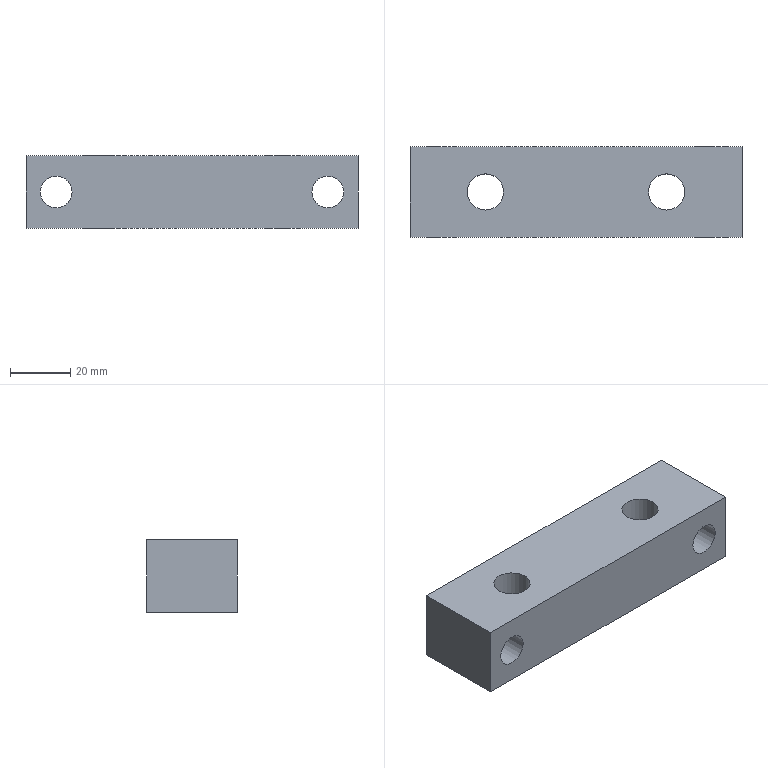Component | NX | SUPPORT_BLOCK | 1 solid | 10 faces | box 110 x 30 x 24 mm | volume 68576 mm3 | plane 6 | cylinder 4 | commonest cylinder face diameters 12 x2 10.5 x2
STEP:
#1=CARTESIAN_POINT('',(0.,0.,0.));
#2=DIRECTION('',(0.,0.,1.));
#3=DIRECTION('',(1.,0.,0.));
#4=AXIS2_PLACEMENT_3D('',#1,#2,#3);
#5=CARTESIAN_POINT('',(-25.,-15.,225.));
#6=VERTEX_POINT('',#5);
#7=CARTESIAN_POINT('',(-25.,15.,225.));
#8=VERTEX_POINT('',#7);
#9=CARTESIAN_POINT('',(-25.,-15.,225.));
#10=DIRECTION('',(0.,1.,0.));
#11=VECTOR('',#10,1.);
#12=LINE('',#9,#11);
#13=CARTESIAN_POINT('',(-25.,-15.,201.));
#14=DIRECTION('',(1.,0.,0.));
#15=DIRECTION('',(0.,1.,0.));
#16=AXIS2_PLACEMENT_3D('',#13,#14,#15);
#17=PLANE('',#16);
#18=CARTESIAN_POINT('',(0.,24.));
#19=DIRECTION('',(1.,0.));
#20=VECTOR('',#19,1.);
#21=LINE('',#18,#20);
#22=(GEOMETRIC_REPRESENTATION_CONTEXT(2)PARAMETRIC_REPRESENTATION_CONTEXT()REPRESENTATION_CONTEXT('',''));
#23=DEFINITIONAL_REPRESENTATION('',(#21),#22);
#24=PCURVE('',#17,#23);
#25=CARTESIAN_POINT('',(0.,0.,225.));
#26=DIRECTION('',(0.,0.,1.));
#27=DIRECTION('',(0.,-1.,0.));
#28=AXIS2_PLACEMENT_3D('',#25,#26,#27);
#29=PLANE('',#28);
#30=CARTESIAN_POINT('',(15.,-25.));
#31=DIRECTION('',(-1.,0.));
#32=VECTOR('',#31,1.);
#33=LINE('',#30,#32);
#34=(GEOMETRIC_REPRESENTATION_CONTEXT(2)PARAMETRIC_REPRESENTATION_CONTEXT()REPRESENTATION_CONTEXT('',''));
#35=DEFINITIONAL_REPRESENTATION('',(#33),#34);
#36=PCURVE('',#29,#35);
#37=SURFACE_CURVE('',#12,(#24,#36),.PCURVE_S1.);
#38=EDGE_CURVE('',#6,#8,#37,.T.);
#39=ORIENTED_EDGE('',*,*,#38,.T.);
#40=CARTESIAN_POINT('',(-25.,15.,201.));
#41=VERTEX_POINT('',#40);
#42=CARTESIAN_POINT('',(-25.,15.,201.));
#43=DIRECTION('',(0.,0.,1.));
#44=VECTOR('',#43,1.);
#45=LINE('',#42,#44);
#46=CARTESIAN_POINT('',(30.,0.));
#47=DIRECTION('',(0.,1.));
#48=VECTOR('',#47,1.);
#49=LINE('',#46,#48);
#50=(GEOMETRIC_REPRESENTATION_CONTEXT(2)PARAMETRIC_REPRESENTATION_CONTEXT()REPRESENTATION_CONTEXT('',''));
#51=DEFINITIONAL_REPRESENTATION('',(#49),#50);
#52=PCURVE('',#17,#51);
#53=CARTESIAN_POINT('',(-25.,15.,201.));
#54=DIRECTION('',(0.,-1.,0.));
#55=DIRECTION('',(1.,0.,0.));
#56=AXIS2_PLACEMENT_3D('',#53,#54,#55);
#57=PLANE('',#56);
#58=CARTESIAN_POINT('',(0.,0.));
#59=DIRECTION('',(0.,1.));
#60=VECTOR('',#59,1.);
#61=LINE('',#58,#60);
#62=(GEOMETRIC_REPRESENTATION_CONTEXT(2)PARAMETRIC_REPRESENTATION_CONTEXT()REPRESENTATION_CONTEXT('',''));
#63=DEFINITIONAL_REPRESENTATION('',(#61),#62);
#64=PCURVE('',#57,#63);
#65=SURFACE_CURVE('',#45,(#52,#64),.PCURVE_S1.);
#66=EDGE_CURVE('',#41,#8,#65,.T.);
#67=ORIENTED_EDGE('',*,*,#66,.F.);
#68=CARTESIAN_POINT('',(-25.,-15.,201.));
#69=VERTEX_POINT('',#68);
#70=CARTESIAN_POINT('',(-25.,-15.,201.));
#71=DIRECTION('',(0.,1.,0.));
#72=VECTOR('',#71,1.);
#73=LINE('',#70,#72);
#74=CARTESIAN_POINT('',(0.,0.));
#75=DIRECTION('',(1.,0.));
#76=VECTOR('',#75,1.);
#77=LINE('',#74,#76);
#78=(GEOMETRIC_REPRESENTATION_CONTEXT(2)PARAMETRIC_REPRESENTATION_CONTEXT()REPRESENTATION_CONTEXT('',''));
#79=DEFINITIONAL_REPRESENTATION('',(#77),#78);
#80=PCURVE('',#17,#79);
#81=CARTESIAN_POINT('',(0.,0.,201.));
#82=DIRECTION('',(0.,0.,1.));
#83=DIRECTION('',(0.,-1.,0.));
#84=AXIS2_PLACEMENT_3D('',#81,#82,#83);
#85=PLANE('',#84);
#86=CARTESIAN_POINT('',(15.,-25.));
#87=DIRECTION('',(-1.,0.));
#88=VECTOR('',#87,1.);
#89=LINE('',#86,#88);
#90=(GEOMETRIC_REPRESENTATION_CONTEXT(2)PARAMETRIC_REPRESENTATION_CONTEXT()REPRESENTATION_CONTEXT('',''));
#91=DEFINITIONAL_REPRESENTATION('',(#89),#90);
#92=PCURVE('',#85,#91);
#93=SURFACE_CURVE('',#73,(#80,#92),.PCURVE_S1.);
#94=EDGE_CURVE('',#69,#41,#93,.T.);
#95=ORIENTED_EDGE('',*,*,#94,.F.);
#96=CARTESIAN_POINT('',(-25.,-15.,201.));
#97=DIRECTION('',(0.,0.,1.));
#98=VECTOR('',#97,1.);
#99=LINE('',#96,#98);
#100=CARTESIAN_POINT('',(0.,0.));
#101=DIRECTION('',(0.,1.));
#102=VECTOR('',#101,1.);
#103=LINE('',#100,#102);
#104=(GEOMETRIC_REPRESENTATION_CONTEXT(2)PARAMETRIC_REPRESENTATION_CONTEXT()REPRESENTATION_CONTEXT('',''));
#105=DEFINITIONAL_REPRESENTATION('',(#103),#104);
#106=PCURVE('',#17,#105);
#107=CARTESIAN_POINT('',(85.,-15.,201.));
#108=DIRECTION('',(-0.,1.,0.));
#109=DIRECTION('',(-1.,-0.,0.));
#110=AXIS2_PLACEMENT_3D('',#107,#108,#109);
#111=PLANE('',#110);
#112=CARTESIAN_POINT('',(110.,0.));
#113=DIRECTION('',(0.,1.));
#114=VECTOR('',#113,1.);
#115=LINE('',#112,#114);
#116=(GEOMETRIC_REPRESENTATION_CONTEXT(2)PARAMETRIC_REPRESENTATION_CONTEXT()REPRESENTATION_CONTEXT('',''));
#117=DEFINITIONAL_REPRESENTATION('',(#115),#116);
#118=PCURVE('',#111,#117);
#119=SURFACE_CURVE('',#99,(#106,#118),.PCURVE_S1.);
#120=EDGE_CURVE('',#69,#6,#119,.T.);
#121=ORIENTED_EDGE('',*,*,#120,.T.);
#122=EDGE_LOOP('',(#39,#67,#95,#121));
#123=FACE_BOUND('',#122,.T.);
#124=ADVANCED_FACE('',(#123),#17,.F.);
#125=CARTESIAN_POINT('',(-9.75,15.,213.));
#126=VERTEX_POINT('',#125);
#127=CARTESIAN_POINT('',(-15.,15.,213.));
#128=DIRECTION('',(-0.,1.,0.));
#129=DIRECTION('',(1.,0.,0.));
#130=AXIS2_PLACEMENT_3D('',#127,#128,#129);
#131=CIRCLE('',#130,5.25);
#132=CARTESIAN_POINT('',(15.25,12.));
#133=CARTESIAN_POINT('',(15.25,2.907));
#134=CARTESIAN_POINT('',(7.375,7.453));
#135=CARTESIAN_POINT('',(-0.5,12.));
#136=CARTESIAN_POINT('',(7.375,16.547));
#137=CARTESIAN_POINT('',(15.25,21.093));
#138=CARTESIAN_POINT('',(15.25,12.));
#139=(BOUNDED_CURVE()B_SPLINE_CURVE(2,(#132,#133,#134,#135,#136,#137,#138),.UNSPECIFIED.,.T.,.F.)B_SPLINE_CURVE_WITH_KNOTS((1,2,2,2,2,1),(-2.094,0.,2.094,4.189,6.283,8.378),.UNSPECIFIED.)CURVE()GEOMETRIC_REPRESENTATION_ITEM()RATIONAL_B_SPLINE_CURVE((1.,0.5,1.,0.5,1.,0.5,1.))REPRESENTATION_ITEM(''));
#140=(GEOMETRIC_REPRESENTATION_CONTEXT(2)PARAMETRIC_REPRESENTATION_CONTEXT()REPRESENTATION_CONTEXT('',''));
#141=DEFINITIONAL_REPRESENTATION('',(#139),#140);
#142=PCURVE('',#57,#141);
#143=CARTESIAN_POINT('',(-15.,22.,213.));
#144=DIRECTION('',(0.,-1.,0.));
#145=DIRECTION('',(1.,0.,0.));
#146=AXIS2_PLACEMENT_3D('',#143,#144,#145);
#147=CYLINDRICAL_SURFACE('',#146,5.25);
#148=CARTESIAN_POINT('',(6.283,7.));
#149=DIRECTION('',(-1.,0.));
#150=VECTOR('',#149,1.);
#151=LINE('',#148,#150);
#152=(GEOMETRIC_REPRESENTATION_CONTEXT(2)PARAMETRIC_REPRESENTATION_CONTEXT()REPRESENTATION_CONTEXT('',''));
#153=DEFINITIONAL_REPRESENTATION('',(#151),#152);
#154=PCURVE('',#147,#153);
#155=SURFACE_CURVE('',#131,(#142,#154),.PCURVE_S1.);
#156=EDGE_CURVE('',#126,#126,#155,.T.);
#157=ORIENTED_EDGE('',*,*,#156,.F.);
#158=EDGE_LOOP('',(#157));
#159=FACE_BOUND('',#158,.T.);
#160=CARTESIAN_POINT('',(80.25,15.,213.));
#161=VERTEX_POINT('',#160);
#162=CARTESIAN_POINT('',(75.,15.,213.));
#163=DIRECTION('',(0.,-1.,0.));
#164=DIRECTION('',(1.,0.,0.));
#165=AXIS2_PLACEMENT_3D('',#162,#163,#164);
#166=CIRCLE('',#165,5.25);
#167=CARTESIAN_POINT('',(100.,12.));
#168=DIRECTION('',(1.,0.));
#169=AXIS2_PLACEMENT_2D('',#167,#168);
#170=CIRCLE('',#169,5.25);
#171=(GEOMETRIC_REPRESENTATION_CONTEXT(2)PARAMETRIC_REPRESENTATION_CONTEXT()REPRESENTATION_CONTEXT('',''));
#172=DEFINITIONAL_REPRESENTATION('',(#170),#171);
#173=PCURVE('',#57,#172);
#174=CARTESIAN_POINT('',(75.,22.,213.));
#175=DIRECTION('',(0.,-1.,0.));
#176=DIRECTION('',(1.,0.,0.));
#177=AXIS2_PLACEMENT_3D('',#174,#175,#176);
#178=CYLINDRICAL_SURFACE('',#177,5.25);
#179=CARTESIAN_POINT('',(0.,7.));
#180=DIRECTION('',(1.,0.));
#181=VECTOR('',#180,1.);
#182=LINE('',#179,#181);
#183=(GEOMETRIC_REPRESENTATION_CONTEXT(2)PARAMETRIC_REPRESENTATION_CONTEXT()REPRESENTATION_CONTEXT('',''));
#184=DEFINITIONAL_REPRESENTATION('',(#182),#183);
#185=PCURVE('',#178,#184);
#186=SURFACE_CURVE('',#166,(#173,#185),.PCURVE_S1.);
#187=EDGE_CURVE('',#161,#161,#186,.T.);
#188=ORIENTED_EDGE('',*,*,#187,.T.);
#189=EDGE_LOOP('',(#188));
#190=FACE_BOUND('',#189,.T.);
#191=CARTESIAN_POINT('',(85.,15.,225.));
#192=VERTEX_POINT('',#191);
#193=CARTESIAN_POINT('',(-25.,15.,225.));
#194=DIRECTION('',(1.,0.,0.));
#195=VECTOR('',#194,1.);
#196=LINE('',#193,#195);
#197=CARTESIAN_POINT('',(0.,24.));
#198=DIRECTION('',(1.,0.));
#199=VECTOR('',#198,1.);
#200=LINE('',#197,#199);
#201=(GEOMETRIC_REPRESENTATION_CONTEXT(2)PARAMETRIC_REPRESENTATION_CONTEXT()REPRESENTATION_CONTEXT('',''));
#202=DEFINITIONAL_REPRESENTATION('',(#200),#201);
#203=PCURVE('',#57,#202);
#204=CARTESIAN_POINT('',(-15.,-25.));
#205=DIRECTION('',(-0.,1.));
#206=VECTOR('',#205,1.);
#207=LINE('',#204,#206);
#208=(GEOMETRIC_REPRESENTATION_CONTEXT(2)PARAMETRIC_REPRESENTATION_CONTEXT()REPRESENTATION_CONTEXT('',''));
#209=DEFINITIONAL_REPRESENTATION('',(#207),#208);
#210=PCURVE('',#29,#209);
#211=SURFACE_CURVE('',#196,(#203,#210),.PCURVE_S1.);
#212=EDGE_CURVE('',#8,#192,#211,.T.);
#213=ORIENTED_EDGE('',*,*,#212,.T.);
#214=CARTESIAN_POINT('',(85.,15.,201.));
#215=VERTEX_POINT('',#214);
#216=CARTESIAN_POINT('',(85.,15.,201.));
#217=DIRECTION('',(0.,0.,1.));
#218=VECTOR('',#217,1.);
#219=LINE('',#216,#218);
#220=CARTESIAN_POINT('',(110.,0.));
#221=DIRECTION('',(0.,1.));
#222=VECTOR('',#221,1.);
#223=LINE('',#220,#222);
#224=(GEOMETRIC_REPRESENTATION_CONTEXT(2)PARAMETRIC_REPRESENTATION_CONTEXT()REPRESENTATION_CONTEXT('',''));
#225=DEFINITIONAL_REPRESENTATION('',(#223),#224);
#226=PCURVE('',#57,#225);
#227=CARTESIAN_POINT('',(85.,15.,201.));
#228=DIRECTION('',(-1.,-0.,0.));
#229=DIRECTION('',(0.,-1.,0.));
#230=AXIS2_PLACEMENT_3D('',#227,#228,#229);
#231=PLANE('',#230);
#232=CARTESIAN_POINT('',(0.,0.));
#233=DIRECTION('',(0.,1.));
#234=VECTOR('',#233,1.);
#235=LINE('',#232,#234);
#236=(GEOMETRIC_REPRESENTATION_CONTEXT(2)PARAMETRIC_REPRESENTATION_CONTEXT()REPRESENTATION_CONTEXT('',''));
#237=DEFINITIONAL_REPRESENTATION('',(#235),#236);
#238=PCURVE('',#231,#237);
#239=SURFACE_CURVE('',#219,(#226,#238),.PCURVE_S1.);
#240=EDGE_CURVE('',#215,#192,#239,.T.);
#241=ORIENTED_EDGE('',*,*,#240,.F.);
#242=CARTESIAN_POINT('',(-25.,15.,201.));
#243=DIRECTION('',(1.,0.,0.));
#244=VECTOR('',#243,1.);
#245=LINE('',#242,#244);
#246=CARTESIAN_POINT('',(0.,0.));
#247=DIRECTION('',(1.,0.));
#248=VECTOR('',#247,1.);
#249=LINE('',#246,#248);
#250=(GEOMETRIC_REPRESENTATION_CONTEXT(2)PARAMETRIC_REPRESENTATION_CONTEXT()REPRESENTATION_CONTEXT('',''));
#251=DEFINITIONAL_REPRESENTATION('',(#249),#250);
#252=PCURVE('',#57,#251);
#253=CARTESIAN_POINT('',(-15.,-25.));
#254=DIRECTION('',(-0.,1.));
#255=VECTOR('',#254,1.);
#256=LINE('',#253,#255);
#257=(GEOMETRIC_REPRESENTATION_CONTEXT(2)PARAMETRIC_REPRESENTATION_CONTEXT()REPRESENTATION_CONTEXT('',''));
#258=DEFINITIONAL_REPRESENTATION('',(#256),#257);
#259=PCURVE('',#85,#258);
#260=SURFACE_CURVE('',#245,(#252,#259),.PCURVE_S1.);
#261=EDGE_CURVE('',#41,#215,#260,.T.);
#262=ORIENTED_EDGE('',*,*,#261,.F.);
#263=ORIENTED_EDGE('',*,*,#66,.T.);
#264=EDGE_LOOP('',(#213,#241,#262,#263));
#265=FACE_BOUND('',#264,.T.);
#266=ADVANCED_FACE('',(#159,#190,#265),#57,.F.);
#267=CARTESIAN_POINT('',(85.,-15.,225.));
#268=VERTEX_POINT('',#267);
#269=CARTESIAN_POINT('',(85.,15.,225.));
#270=DIRECTION('',(0.,-1.,0.));
#271=VECTOR('',#270,1.);
#272=LINE('',#269,#271);
#273=CARTESIAN_POINT('',(0.,24.));
#274=DIRECTION('',(1.,0.));
#275=VECTOR('',#274,1.);
#276=LINE('',#273,#275);
#277=(GEOMETRIC_REPRESENTATION_CONTEXT(2)PARAMETRIC_REPRESENTATION_CONTEXT()REPRESENTATION_CONTEXT('',''));
#278=DEFINITIONAL_REPRESENTATION('',(#276),#277);
#279=PCURVE('',#231,#278);
#280=CARTESIAN_POINT('',(-15.,85.));
#281=DIRECTION('',(1.,0.));
#282=VECTOR('',#281,1.);
#283=LINE('',#280,#282);
#284=(GEOMETRIC_REPRESENTATION_CONTEXT(2)PARAMETRIC_REPRESENTATION_CONTEXT()REPRESENTATION_CONTEXT('',''));
#285=DEFINITIONAL_REPRESENTATION('',(#283),#284);
#286=PCURVE('',#29,#285);
#287=SURFACE_CURVE('',#272,(#279,#286),.PCURVE_S1.);
#288=EDGE_CURVE('',#192,#268,#287,.T.);
#289=ORIENTED_EDGE('',*,*,#288,.T.);
#290=CARTESIAN_POINT('',(85.,-15.,201.));
#291=VERTEX_POINT('',#290);
#292=CARTESIAN_POINT('',(85.,-15.,201.));
#293=DIRECTION('',(0.,0.,1.));
#294=VECTOR('',#293,1.);
#295=LINE('',#292,#294);
#296=CARTESIAN_POINT('',(30.,0.));
#297=DIRECTION('',(0.,1.));
#298=VECTOR('',#297,1.);
#299=LINE('',#296,#298);
#300=(GEOMETRIC_REPRESENTATION_CONTEXT(2)PARAMETRIC_REPRESENTATION_CONTEXT()REPRESENTATION_CONTEXT('',''));
#301=DEFINITIONAL_REPRESENTATION('',(#299),#300);
#302=PCURVE('',#231,#301);
#303=CARTESIAN_POINT('',(0.,0.));
#304=DIRECTION('',(0.,1.));
#305=VECTOR('',#304,1.);
#306=LINE('',#303,#305);
#307=(GEOMETRIC_REPRESENTATION_CONTEXT(2)PARAMETRIC_REPRESENTATION_CONTEXT()REPRESENTATION_CONTEXT('',''));
#308=DEFINITIONAL_REPRESENTATION('',(#306),#307);
#309=PCURVE('',#111,#308);
#310=SURFACE_CURVE('',#295,(#302,#309),.PCURVE_S1.);
#311=EDGE_CURVE('',#291,#268,#310,.T.);
#312=ORIENTED_EDGE('',*,*,#311,.F.);
#313=CARTESIAN_POINT('',(85.,15.,201.));
#314=DIRECTION('',(0.,-1.,0.));
#315=VECTOR('',#314,1.);
#316=LINE('',#313,#315);
#317=CARTESIAN_POINT('',(0.,0.));
#318=DIRECTION('',(1.,0.));
#319=VECTOR('',#318,1.);
#320=LINE('',#317,#319);
#321=(GEOMETRIC_REPRESENTATION_CONTEXT(2)PARAMETRIC_REPRESENTATION_CONTEXT()REPRESENTATION_CONTEXT('',''));
#322=DEFINITIONAL_REPRESENTATION('',(#320),#321);
#323=PCURVE('',#231,#322);
#324=CARTESIAN_POINT('',(-15.,85.));
#325=DIRECTION('',(1.,0.));
#326=VECTOR('',#325,1.);
#327=LINE('',#324,#326);
#328=(GEOMETRIC_REPRESENTATION_CONTEXT(2)PARAMETRIC_REPRESENTATION_CONTEXT()REPRESENTATION_CONTEXT('',''));
#329=DEFINITIONAL_REPRESENTATION('',(#327),#328);
#330=PCURVE('',#85,#329);
#331=SURFACE_CURVE('',#316,(#323,#330),.PCURVE_S1.);
#332=EDGE_CURVE('',#215,#291,#331,.T.);
#333=ORIENTED_EDGE('',*,*,#332,.F.);
#334=ORIENTED_EDGE('',*,*,#240,.T.);
#335=EDGE_LOOP('',(#289,#312,#333,#334));
#336=FACE_BOUND('',#335,.T.);
#337=ADVANCED_FACE('',(#336),#231,.F.);
#338=CARTESIAN_POINT('',(0.,-6.,201.));
#339=VERTEX_POINT('',#338);
#340=CARTESIAN_POINT('',(0.,0.,201.));
#341=DIRECTION('',(0.,0.,1.));
#342=DIRECTION('',(0.,-1.,0.));
#343=AXIS2_PLACEMENT_3D('',#340,#341,#342);
#344=CIRCLE('',#343,6.);
#345=CARTESIAN_POINT('',(0.,0.,201.));
#346=DIRECTION('',(0.,0.,1.));
#347=DIRECTION('',(0.,-1.,0.));
#348=AXIS2_PLACEMENT_3D('',#345,#346,#347);
#349=CYLINDRICAL_SURFACE('',#348,6.);
#350=CARTESIAN_POINT('',(0.,0.));
#351=DIRECTION('',(1.,0.));
#352=VECTOR('',#351,1.);
#353=LINE('',#350,#352);
#354=(GEOMETRIC_REPRESENTATION_CONTEXT(2)PARAMETRIC_REPRESENTATION_CONTEXT()REPRESENTATION_CONTEXT('',''));
#355=DEFINITIONAL_REPRESENTATION('',(#353),#354);
#356=PCURVE('',#349,#355);
#357=CARTESIAN_POINT('',(0.,0.));
#358=DIRECTION('',(1.,0.));
#359=AXIS2_PLACEMENT_2D('',#357,#358);
#360=CIRCLE('',#359,6.);
#361=(GEOMETRIC_REPRESENTATION_CONTEXT(2)PARAMETRIC_REPRESENTATION_CONTEXT()REPRESENTATION_CONTEXT('',''));
#362=DEFINITIONAL_REPRESENTATION('',(#360),#361);
#363=PCURVE('',#85,#362);
#364=SURFACE_CURVE('',#344,(#356,#363),.PCURVE_S1.);
#365=EDGE_CURVE('',#339,#339,#364,.T.);
#366=ORIENTED_EDGE('',*,*,#365,.T.);
#367=CARTESIAN_POINT('',(0.,-6.,225.));
#368=VERTEX_POINT('',#367);
#369=CARTESIAN_POINT('',(0.,-6.,201.));
#370=CARTESIAN_POINT('',(0.,-6.,225.));
#371=B_SPLINE_CURVE_WITH_KNOTS('',1,(#369,#370),.UNSPECIFIED.,.F.,.F.,(2,2),(0.,24.),.PIECEWISE_BEZIER_KNOTS.);
#372=CARTESIAN_POINT('',(6.283,0.));
#373=DIRECTION('',(0.,1.));
#374=VECTOR('',#373,1.);
#375=LINE('',#372,#374);
#376=(GEOMETRIC_REPRESENTATION_CONTEXT(2)PARAMETRIC_REPRESENTATION_CONTEXT()REPRESENTATION_CONTEXT('',''));
#377=DEFINITIONAL_REPRESENTATION('',(#375),#376);
#378=PCURVE('',#349,#377);
#379=CARTESIAN_POINT('',(0.,0.));
#380=DIRECTION('',(0.,1.));
#381=VECTOR('',#380,1.);
#382=LINE('',#379,#381);
#383=(GEOMETRIC_REPRESENTATION_CONTEXT(2)PARAMETRIC_REPRESENTATION_CONTEXT()REPRESENTATION_CONTEXT('',''));
#384=DEFINITIONAL_REPRESENTATION('',(#382),#383);
#385=PCURVE('',#349,#384);
#386=SEAM_CURVE('',#371,(#378,#385),.PCURVE_S1.);
#387=EDGE_CURVE('',#339,#368,#386,.T.);
#388=ORIENTED_EDGE('',*,*,#387,.T.);
#389=CARTESIAN_POINT('',(0.,0.,225.));
#390=DIRECTION('',(0.,0.,1.));
#391=DIRECTION('',(0.,-1.,0.));
#392=AXIS2_PLACEMENT_3D('',#389,#390,#391);
#393=CIRCLE('',#392,6.);
#394=CARTESIAN_POINT('',(0.,24.));
#395=DIRECTION('',(1.,0.));
#396=VECTOR('',#395,1.);
#397=LINE('',#394,#396);
#398=(GEOMETRIC_REPRESENTATION_CONTEXT(2)PARAMETRIC_REPRESENTATION_CONTEXT()REPRESENTATION_CONTEXT('',''));
#399=DEFINITIONAL_REPRESENTATION('',(#397),#398);
#400=PCURVE('',#349,#399);
#401=CARTESIAN_POINT('',(0.,0.));
#402=DIRECTION('',(1.,0.));
#403=AXIS2_PLACEMENT_2D('',#401,#402);
#404=CIRCLE('',#403,6.);
#405=(GEOMETRIC_REPRESENTATION_CONTEXT(2)PARAMETRIC_REPRESENTATION_CONTEXT()REPRESENTATION_CONTEXT('',''));
#406=DEFINITIONAL_REPRESENTATION('',(#404),#405);
#407=PCURVE('',#29,#406);
#408=SURFACE_CURVE('',#393,(#400,#407),.PCURVE_S1.);
#409=EDGE_CURVE('',#368,#368,#408,.T.);
#410=ORIENTED_EDGE('',*,*,#409,.F.);
#411=ORIENTED_EDGE('',*,*,#387,.F.);
#412=EDGE_LOOP('',(#366,#388,#410,#411));
#413=FACE_BOUND('',#412,.F.);
#414=ADVANCED_FACE('',(#413),#349,.F.);
#415=CARTESIAN_POINT('',(-9.75,-15.,213.));
#416=VERTEX_POINT('',#415);
#417=CARTESIAN_POINT('',(-15.,-15.,213.));
#418=DIRECTION('',(0.,1.,0.));
#419=DIRECTION('',(1.,0.,0.));
#420=AXIS2_PLACEMENT_3D('',#417,#418,#419);
#421=CIRCLE('',#420,5.25);
#422=CARTESIAN_POINT('',(100.,12.));
#423=DIRECTION('',(-1.,0.));
#424=AXIS2_PLACEMENT_2D('',#422,#423);
#425=CIRCLE('',#424,5.25);
#426=(GEOMETRIC_REPRESENTATION_CONTEXT(2)PARAMETRIC_REPRESENTATION_CONTEXT()REPRESENTATION_CONTEXT('',''));
#427=DEFINITIONAL_REPRESENTATION('',(#425),#426);
#428=PCURVE('',#111,#427);
#429=CARTESIAN_POINT('',(6.283,37.));
#430=DIRECTION('',(-1.,0.));
#431=VECTOR('',#430,1.);
#432=LINE('',#429,#431);
#433=(GEOMETRIC_REPRESENTATION_CONTEXT(2)PARAMETRIC_REPRESENTATION_CONTEXT()REPRESENTATION_CONTEXT('',''));
#434=DEFINITIONAL_REPRESENTATION('',(#432),#433);
#435=PCURVE('',#147,#434);
#436=SURFACE_CURVE('',#421,(#428,#435),.PCURVE_S1.);
#437=EDGE_CURVE('',#416,#416,#436,.T.);
#438=ORIENTED_EDGE('',*,*,#437,.T.);
#439=EDGE_LOOP('',(#438));
#440=FACE_BOUND('',#439,.T.);
#441=CARTESIAN_POINT('',(69.75,-15.,213.));
#442=VERTEX_POINT('',#441);
#443=CARTESIAN_POINT('',(80.25,-15.,213.));
#444=VERTEX_POINT('',#443);
#445=CARTESIAN_POINT('',(75.,-15.,213.));
#446=DIRECTION('',(0.,-1.,0.));
#447=DIRECTION('',(-1.,0.,0.));
#448=AXIS2_PLACEMENT_3D('',#445,#446,#447);
#449=CIRCLE('',#448,5.25);
#450=CARTESIAN_POINT('',(15.25,12.));
#451=CARTESIAN_POINT('',(15.25,2.907));
#452=CARTESIAN_POINT('',(7.375,7.453));
#453=CARTESIAN_POINT('',(-0.5,12.));
#454=CARTESIAN_POINT('',(7.375,16.547));
#455=CARTESIAN_POINT('',(15.25,21.093));
#456=CARTESIAN_POINT('',(15.25,12.));
#457=(BOUNDED_CURVE()B_SPLINE_CURVE(2,(#450,#451,#452,#453,#454,#455,#456),.UNSPECIFIED.,.T.,.F.)B_SPLINE_CURVE_WITH_KNOTS((1,2,2,2,2,1),(-2.094,0.,2.094,4.189,6.283,8.378),.UNSPECIFIED.)CURVE()GEOMETRIC_REPRESENTATION_ITEM()RATIONAL_B_SPLINE_CURVE((1.,0.5,1.,0.5,1.,0.5,1.))REPRESENTATION_ITEM(''));
#458=(GEOMETRIC_REPRESENTATION_CONTEXT(2)PARAMETRIC_REPRESENTATION_CONTEXT()REPRESENTATION_CONTEXT('',''));
#459=DEFINITIONAL_REPRESENTATION('',(#457),#458);
#460=PCURVE('',#111,#459);
#461=CARTESIAN_POINT('',(3.142,37.));
#462=DIRECTION('',(1.,0.));
#463=VECTOR('',#462,1.);
#464=LINE('',#461,#463);
#465=(GEOMETRIC_REPRESENTATION_CONTEXT(2)PARAMETRIC_REPRESENTATION_CONTEXT()REPRESENTATION_CONTEXT('',''));
#466=DEFINITIONAL_REPRESENTATION('',(#464),#465);
#467=PCURVE('',#178,#466);
#468=SURFACE_CURVE('',#449,(#460,#467),.PCURVE_S1.);
#469=EDGE_CURVE('',#442,#444,#468,.T.);
#470=ORIENTED_EDGE('',*,*,#469,.F.);
#471=CARTESIAN_POINT('',(75.,-15.,213.));
#472=DIRECTION('',(0.,-1.,0.));
#473=DIRECTION('',(-1.,0.,0.));
#474=AXIS2_PLACEMENT_3D('',#471,#472,#473);
#475=CIRCLE('',#474,5.25);
#476=CARTESIAN_POINT('',(15.25,12.));
#477=CARTESIAN_POINT('',(15.25,2.907));
#478=CARTESIAN_POINT('',(7.375,7.453));
#479=CARTESIAN_POINT('',(-0.5,12.));
#480=CARTESIAN_POINT('',(7.375,16.547));
#481=CARTESIAN_POINT('',(15.25,21.093));
#482=CARTESIAN_POINT('',(15.25,12.));
#483=(BOUNDED_CURVE()B_SPLINE_CURVE(2,(#476,#477,#478,#479,#480,#481,#482),.UNSPECIFIED.,.T.,.F.)B_SPLINE_CURVE_WITH_KNOTS((1,2,2,2,2,1),(-2.094,0.,2.094,4.189,6.283,8.378),.UNSPECIFIED.)CURVE()GEOMETRIC_REPRESENTATION_ITEM()RATIONAL_B_SPLINE_CURVE((1.,0.5,1.,0.5,1.,0.5,1.))REPRESENTATION_ITEM(''));
#484=(GEOMETRIC_REPRESENTATION_CONTEXT(2)PARAMETRIC_REPRESENTATION_CONTEXT()REPRESENTATION_CONTEXT('',''));
#485=DEFINITIONAL_REPRESENTATION('',(#483),#484);
#486=PCURVE('',#111,#485);
#487=CARTESIAN_POINT('',(-3.142,37.));
#488=DIRECTION('',(1.,0.));
#489=VECTOR('',#488,1.);
#490=LINE('',#487,#489);
#491=(GEOMETRIC_REPRESENTATION_CONTEXT(2)PARAMETRIC_REPRESENTATION_CONTEXT()REPRESENTATION_CONTEXT('',''));
#492=DEFINITIONAL_REPRESENTATION('',(#490),#491);
#493=PCURVE('',#178,#492);
#494=SURFACE_CURVE('',#475,(#486,#493),.PCURVE_S1.);
#495=EDGE_CURVE('',#444,#442,#494,.T.);
#496=ORIENTED_EDGE('',*,*,#495,.F.);
#497=EDGE_LOOP('',(#470,#496));
#498=FACE_BOUND('',#497,.T.);
#499=CARTESIAN_POINT('',(85.,-15.,225.));
#500=DIRECTION('',(-1.,-0.,0.));
#501=VECTOR('',#500,1.);
#502=LINE('',#499,#501);
#503=CARTESIAN_POINT('',(0.,24.));
#504=DIRECTION('',(1.,0.));
#505=VECTOR('',#504,1.);
#506=LINE('',#503,#505);
#507=(GEOMETRIC_REPRESENTATION_CONTEXT(2)PARAMETRIC_REPRESENTATION_CONTEXT()REPRESENTATION_CONTEXT('',''));
#508=DEFINITIONAL_REPRESENTATION('',(#506),#507);
#509=PCURVE('',#111,#508);
#510=CARTESIAN_POINT('',(15.,85.));
#511=DIRECTION('',(0.,-1.));
#512=VECTOR('',#511,1.);
#513=LINE('',#510,#512);
#514=(GEOMETRIC_REPRESENTATION_CONTEXT(2)PARAMETRIC_REPRESENTATION_CONTEXT()REPRESENTATION_CONTEXT('',''));
#515=DEFINITIONAL_REPRESENTATION('',(#513),#514);
#516=PCURVE('',#29,#515);
#517=SURFACE_CURVE('',#502,(#509,#516),.PCURVE_S1.);
#518=EDGE_CURVE('',#268,#6,#517,.T.);
#519=ORIENTED_EDGE('',*,*,#518,.T.);
#520=ORIENTED_EDGE('',*,*,#120,.F.);
#521=CARTESIAN_POINT('',(85.,-15.,201.));
#522=DIRECTION('',(-1.,-0.,0.));
#523=VECTOR('',#522,1.);
#524=LINE('',#521,#523);
#525=CARTESIAN_POINT('',(0.,0.));
#526=DIRECTION('',(1.,0.));
#527=VECTOR('',#526,1.);
#528=LINE('',#525,#527);
#529=(GEOMETRIC_REPRESENTATION_CONTEXT(2)PARAMETRIC_REPRESENTATION_CONTEXT()REPRESENTATION_CONTEXT('',''));
#530=DEFINITIONAL_REPRESENTATION('',(#528),#529);
#531=PCURVE('',#111,#530);
#532=CARTESIAN_POINT('',(15.,85.));
#533=DIRECTION('',(0.,-1.));
#534=VECTOR('',#533,1.);
#535=LINE('',#532,#534);
#536=(GEOMETRIC_REPRESENTATION_CONTEXT(2)PARAMETRIC_REPRESENTATION_CONTEXT()REPRESENTATION_CONTEXT('',''));
#537=DEFINITIONAL_REPRESENTATION('',(#535),#536);
#538=PCURVE('',#85,#537);
#539=SURFACE_CURVE('',#524,(#531,#538),.PCURVE_S1.);
#540=EDGE_CURVE('',#291,#69,#539,.T.);
#541=ORIENTED_EDGE('',*,*,#540,.F.);
#542=ORIENTED_EDGE('',*,*,#311,.T.);
#543=EDGE_LOOP('',(#519,#520,#541,#542));
#544=FACE_BOUND('',#543,.T.);
#545=ADVANCED_FACE('',(#440,#498,#544),#111,.F.);
#546=CARTESIAN_POINT('',(60.,-6.,201.));
#547=VERTEX_POINT('',#546);
#548=CARTESIAN_POINT('',(60.,0.,201.));
#549=DIRECTION('',(0.,0.,-1.));
#550=DIRECTION('',(0.,-1.,0.));
#551=AXIS2_PLACEMENT_3D('',#548,#549,#550);
#552=CIRCLE('',#551,6.);
#553=CARTESIAN_POINT('',(60.,0.,201.));
#554=DIRECTION('',(0.,0.,1.));
#555=DIRECTION('',(0.,-1.,0.));
#556=AXIS2_PLACEMENT_3D('',#553,#554,#555);
#557=CYLINDRICAL_SURFACE('',#556,6.);
#558=CARTESIAN_POINT('',(6.283,0.));
#559=DIRECTION('',(-1.,0.));
#560=VECTOR('',#559,1.);
#561=LINE('',#558,#560);
#562=(GEOMETRIC_REPRESENTATION_CONTEXT(2)PARAMETRIC_REPRESENTATION_CONTEXT()REPRESENTATION_CONTEXT('',''));
#563=DEFINITIONAL_REPRESENTATION('',(#561),#562);
#564=PCURVE('',#557,#563);
#565=CARTESIAN_POINT('',(6.,60.));
#566=CARTESIAN_POINT('',(6.,49.608));
#567=CARTESIAN_POINT('',(-3.,54.804));
#568=CARTESIAN_POINT('',(-12.,60.));
#569=CARTESIAN_POINT('',(-3.,65.196));
#570=CARTESIAN_POINT('',(6.,70.392));
#571=CARTESIAN_POINT('',(6.,60.));
#572=(BOUNDED_CURVE()B_SPLINE_CURVE(2,(#565,#566,#567,#568,#569,#570,#571),.UNSPECIFIED.,.T.,.F.)B_SPLINE_CURVE_WITH_KNOTS((1,2,2,2,2,1),(-2.094,0.,2.094,4.189,6.283,8.378),.UNSPECIFIED.)CURVE()GEOMETRIC_REPRESENTATION_ITEM()RATIONAL_B_SPLINE_CURVE((1.,0.5,1.,0.5,1.,0.5,1.))REPRESENTATION_ITEM(''));
#573=(GEOMETRIC_REPRESENTATION_CONTEXT(2)PARAMETRIC_REPRESENTATION_CONTEXT()REPRESENTATION_CONTEXT('',''));
#574=DEFINITIONAL_REPRESENTATION('',(#572),#573);
#575=PCURVE('',#85,#574);
#576=SURFACE_CURVE('',#552,(#564,#575),.PCURVE_S1.);
#577=EDGE_CURVE('',#547,#547,#576,.T.);
#578=ORIENTED_EDGE('',*,*,#577,.F.);
#579=CARTESIAN_POINT('',(60.,-6.,225.));
#580=VERTEX_POINT('',#579);
#581=CARTESIAN_POINT('',(60.,-6.,201.));
#582=CARTESIAN_POINT('',(60.,-6.,225.));
#583=B_SPLINE_CURVE_WITH_KNOTS('',1,(#581,#582),.UNSPECIFIED.,.F.,.F.,(2,2),(0.,24.),.PIECEWISE_BEZIER_KNOTS.);
#584=CARTESIAN_POINT('',(6.283,0.));
#585=DIRECTION('',(0.,1.));
#586=VECTOR('',#585,1.);
#587=LINE('',#584,#586);
#588=(GEOMETRIC_REPRESENTATION_CONTEXT(2)PARAMETRIC_REPRESENTATION_CONTEXT()REPRESENTATION_CONTEXT('',''));
#589=DEFINITIONAL_REPRESENTATION('',(#587),#588);
#590=PCURVE('',#557,#589);
#591=CARTESIAN_POINT('',(0.,0.));
#592=DIRECTION('',(0.,1.));
#593=VECTOR('',#592,1.);
#594=LINE('',#591,#593);
#595=(GEOMETRIC_REPRESENTATION_CONTEXT(2)PARAMETRIC_REPRESENTATION_CONTEXT()REPRESENTATION_CONTEXT('',''));
#596=DEFINITIONAL_REPRESENTATION('',(#594),#595);
#597=PCURVE('',#557,#596);
#598=SEAM_CURVE('',#583,(#590,#597),.PCURVE_S1.);
#599=EDGE_CURVE('',#547,#580,#598,.T.);
#600=ORIENTED_EDGE('',*,*,#599,.T.);
#601=CARTESIAN_POINT('',(60.,0.,225.));
#602=DIRECTION('',(0.,0.,-1.));
#603=DIRECTION('',(0.,-1.,0.));
#604=AXIS2_PLACEMENT_3D('',#601,#602,#603);
#605=CIRCLE('',#604,6.);
#606=CARTESIAN_POINT('',(6.283,24.));
#607=DIRECTION('',(-1.,0.));
#608=VECTOR('',#607,1.);
#609=LINE('',#606,#608);
#610=(GEOMETRIC_REPRESENTATION_CONTEXT(2)PARAMETRIC_REPRESENTATION_CONTEXT()REPRESENTATION_CONTEXT('',''));
#611=DEFINITIONAL_REPRESENTATION('',(#609),#610);
#612=PCURVE('',#557,#611);
#613=CARTESIAN_POINT('',(6.,60.));
#614=CARTESIAN_POINT('',(6.,49.608));
#615=CARTESIAN_POINT('',(-3.,54.804));
#616=CARTESIAN_POINT('',(-12.,60.));
#617=CARTESIAN_POINT('',(-3.,65.196));
#618=CARTESIAN_POINT('',(6.,70.392));
#619=CARTESIAN_POINT('',(6.,60.));
#620=(BOUNDED_CURVE()B_SPLINE_CURVE(2,(#613,#614,#615,#616,#617,#618,#619),.UNSPECIFIED.,.T.,.F.)B_SPLINE_CURVE_WITH_KNOTS((1,2,2,2,2,1),(-2.094,0.,2.094,4.189,6.283,8.378),.UNSPECIFIED.)CURVE()GEOMETRIC_REPRESENTATION_ITEM()RATIONAL_B_SPLINE_CURVE((1.,0.5,1.,0.5,1.,0.5,1.))REPRESENTATION_ITEM(''));
#621=(GEOMETRIC_REPRESENTATION_CONTEXT(2)PARAMETRIC_REPRESENTATION_CONTEXT()REPRESENTATION_CONTEXT('',''));
#622=DEFINITIONAL_REPRESENTATION('',(#620),#621);
#623=PCURVE('',#29,#622);
#624=SURFACE_CURVE('',#605,(#612,#623),.PCURVE_S1.);
#625=EDGE_CURVE('',#580,#580,#624,.T.);
#626=ORIENTED_EDGE('',*,*,#625,.T.);
#627=ORIENTED_EDGE('',*,*,#599,.F.);
#628=EDGE_LOOP('',(#578,#600,#626,#627));
#629=FACE_BOUND('',#628,.F.);
#630=ADVANCED_FACE('',(#629),#557,.F.);
#631=ORIENTED_EDGE('',*,*,#94,.T.);
#632=ORIENTED_EDGE('',*,*,#261,.T.);
#633=ORIENTED_EDGE('',*,*,#332,.T.);
#634=ORIENTED_EDGE('',*,*,#540,.T.);
#635=EDGE_LOOP('',(#631,#632,#633,#634));
#636=FACE_BOUND('',#635,.T.);
#637=ORIENTED_EDGE('',*,*,#365,.T.);
#638=EDGE_LOOP('',(#637));
#639=FACE_BOUND('',#638,.T.);
#640=ORIENTED_EDGE('',*,*,#577,.F.);
#641=EDGE_LOOP('',(#640));
#642=FACE_BOUND('',#641,.T.);
#643=ADVANCED_FACE('',(#636,#639,#642),#85,.F.);
#644=ORIENTED_EDGE('',*,*,#38,.F.);
#645=ORIENTED_EDGE('',*,*,#518,.F.);
#646=ORIENTED_EDGE('',*,*,#288,.F.);
#647=ORIENTED_EDGE('',*,*,#212,.F.);
#648=EDGE_LOOP('',(#644,#645,#646,#647));
#649=FACE_BOUND('',#648,.T.);
#650=ORIENTED_EDGE('',*,*,#409,.F.);
#651=EDGE_LOOP('',(#650));
#652=FACE_BOUND('',#651,.T.);
#653=ORIENTED_EDGE('',*,*,#625,.T.);
#654=EDGE_LOOP('',(#653));
#655=FACE_BOUND('',#654,.T.);
#656=ADVANCED_FACE('',(#649,#652,#655),#29,.T.);
#657=ORIENTED_EDGE('',*,*,#495,.F.);
#658=CARTESIAN_POINT('',(80.25,15.,213.));
#659=CARTESIAN_POINT('',(80.25,-15.,213.));
#660=B_SPLINE_CURVE_WITH_KNOTS('',1,(#658,#659),.UNSPECIFIED.,.F.,.F.,(2,2),(7.,37.),.PIECEWISE_BEZIER_KNOTS.);
#661=CARTESIAN_POINT('',(0.,0.));
#662=DIRECTION('',(0.,1.));
#663=VECTOR('',#662,1.);
#664=LINE('',#661,#663);
#665=(GEOMETRIC_REPRESENTATION_CONTEXT(2)PARAMETRIC_REPRESENTATION_CONTEXT()REPRESENTATION_CONTEXT('',''));
#666=DEFINITIONAL_REPRESENTATION('',(#664),#665);
#667=PCURVE('',#178,#666);
#668=CARTESIAN_POINT('',(6.283,0.));
#669=DIRECTION('',(0.,1.));
#670=VECTOR('',#669,1.);
#671=LINE('',#668,#670);
#672=(GEOMETRIC_REPRESENTATION_CONTEXT(2)PARAMETRIC_REPRESENTATION_CONTEXT()REPRESENTATION_CONTEXT('',''));
#673=DEFINITIONAL_REPRESENTATION('',(#671),#672);
#674=PCURVE('',#178,#673);
#675=SEAM_CURVE('',#660,(#667,#674),.PCURVE_S1.);
#676=EDGE_CURVE('',#161,#444,#675,.T.);
#677=ORIENTED_EDGE('',*,*,#676,.F.);
#678=ORIENTED_EDGE('',*,*,#187,.T.);
#679=ORIENTED_EDGE('',*,*,#676,.T.);
#680=ORIENTED_EDGE('',*,*,#469,.F.);
#681=EDGE_LOOP('',(#657,#677,#678,#679,#680));
#682=FACE_BOUND('',#681,.F.);
#683=ADVANCED_FACE('',(#682),#178,.F.);
#684=ORIENTED_EDGE('',*,*,#437,.T.);
#685=CARTESIAN_POINT('',(-9.75,15.,213.));
#686=CARTESIAN_POINT('',(-9.75,-15.,213.));
#687=B_SPLINE_CURVE_WITH_KNOTS('',1,(#685,#686),.UNSPECIFIED.,.F.,.F.,(2,2),(7.,37.),.PIECEWISE_BEZIER_KNOTS.);
#688=CARTESIAN_POINT('',(0.,0.));
#689=DIRECTION('',(0.,1.));
#690=VECTOR('',#689,1.);
#691=LINE('',#688,#690);
#692=(GEOMETRIC_REPRESENTATION_CONTEXT(2)PARAMETRIC_REPRESENTATION_CONTEXT()REPRESENTATION_CONTEXT('',''));
#693=DEFINITIONAL_REPRESENTATION('',(#691),#692);
#694=PCURVE('',#147,#693);
#695=CARTESIAN_POINT('',(6.283,0.));
#696=DIRECTION('',(0.,1.));
#697=VECTOR('',#696,1.);
#698=LINE('',#695,#697);
#699=(GEOMETRIC_REPRESENTATION_CONTEXT(2)PARAMETRIC_REPRESENTATION_CONTEXT()REPRESENTATION_CONTEXT('',''));
#700=DEFINITIONAL_REPRESENTATION('',(#698),#699);
#701=PCURVE('',#147,#700);
#702=SEAM_CURVE('',#687,(#694,#701),.PCURVE_S1.);
#703=EDGE_CURVE('',#126,#416,#702,.T.);
#704=ORIENTED_EDGE('',*,*,#703,.F.);
#705=ORIENTED_EDGE('',*,*,#156,.F.);
#706=ORIENTED_EDGE('',*,*,#703,.T.);
#707=EDGE_LOOP('',(#684,#704,#705,#706));
#708=FACE_BOUND('',#707,.F.);
#709=ADVANCED_FACE('',(#708),#147,.F.);
#710=CLOSED_SHELL('',(#124,#266,#337,#414,#545,#630,#643,#656,#683,#709));
#711=MANIFOLD_SOLID_BREP('',#710);
#712=(LENGTH_UNIT()NAMED_UNIT(*)SI_UNIT(.MILLI.,.METRE.));
#713=UNCERTAINTY_MEASURE_WITH_UNIT(LENGTH_MEASURE(0.000005),#712,'','');
#714=(NAMED_UNIT(*)PLANE_ANGLE_UNIT()SI_UNIT($,.RADIAN.));
#715=(NAMED_UNIT(*)SI_UNIT($,.STERADIAN.)SOLID_ANGLE_UNIT());
#716=(GEOMETRIC_REPRESENTATION_CONTEXT(3)GLOBAL_UNCERTAINTY_ASSIGNED_CONTEXT((#713))GLOBAL_UNIT_ASSIGNED_CONTEXT((#712,#714,#715))REPRESENTATION_CONTEXT('',''));
#717=ADVANCED_BREP_SHAPE_REPRESENTATION('',(#4,#711),#716);